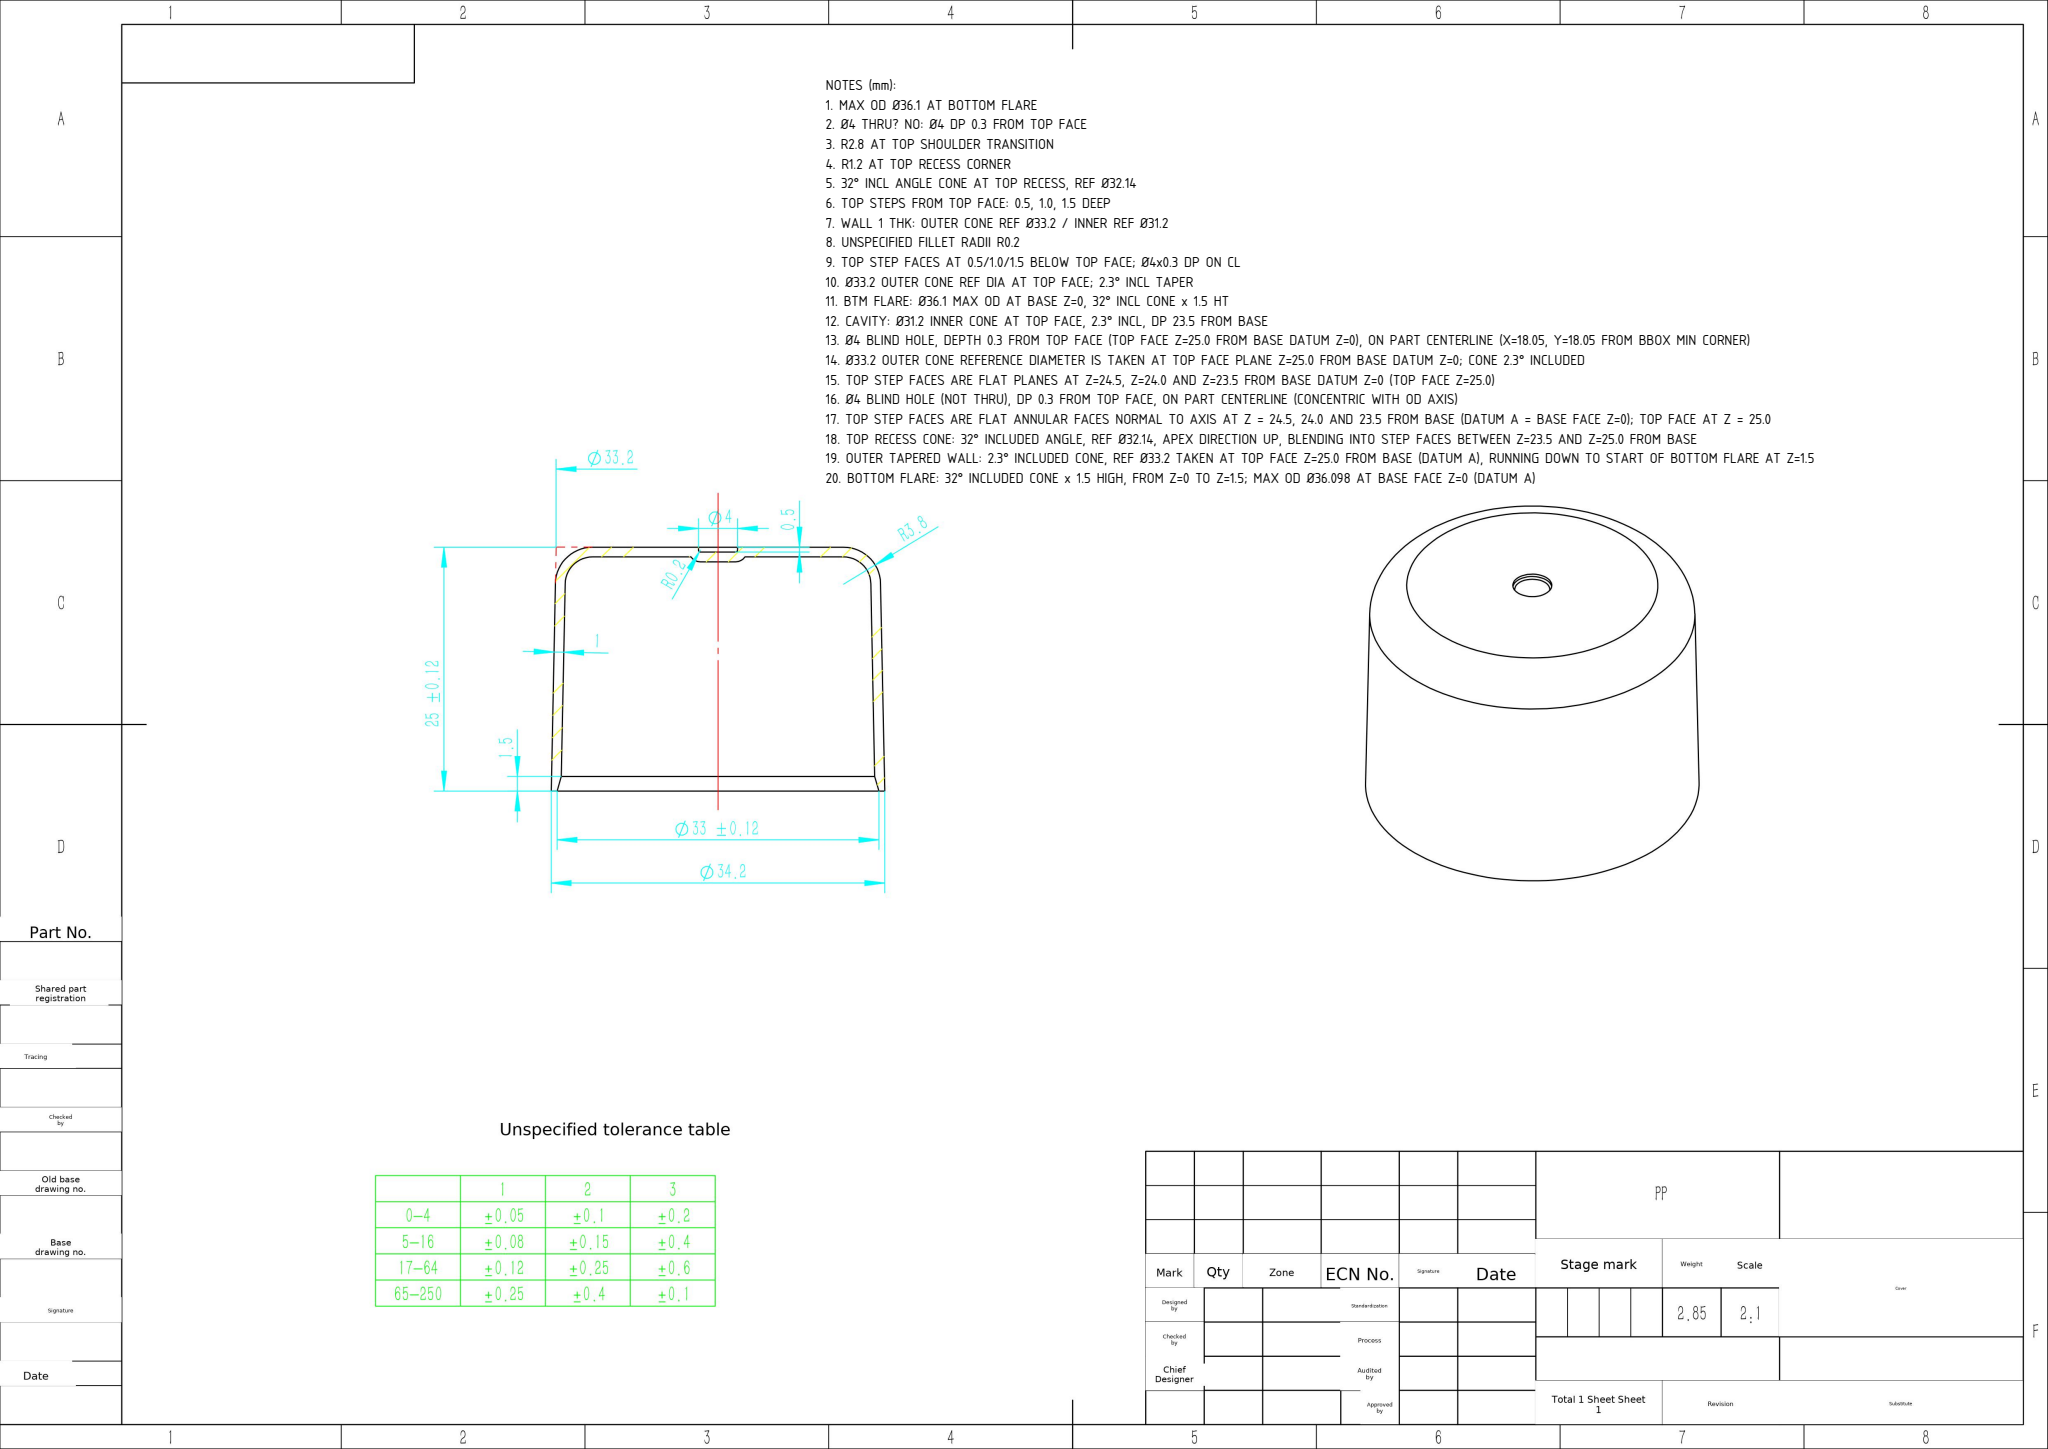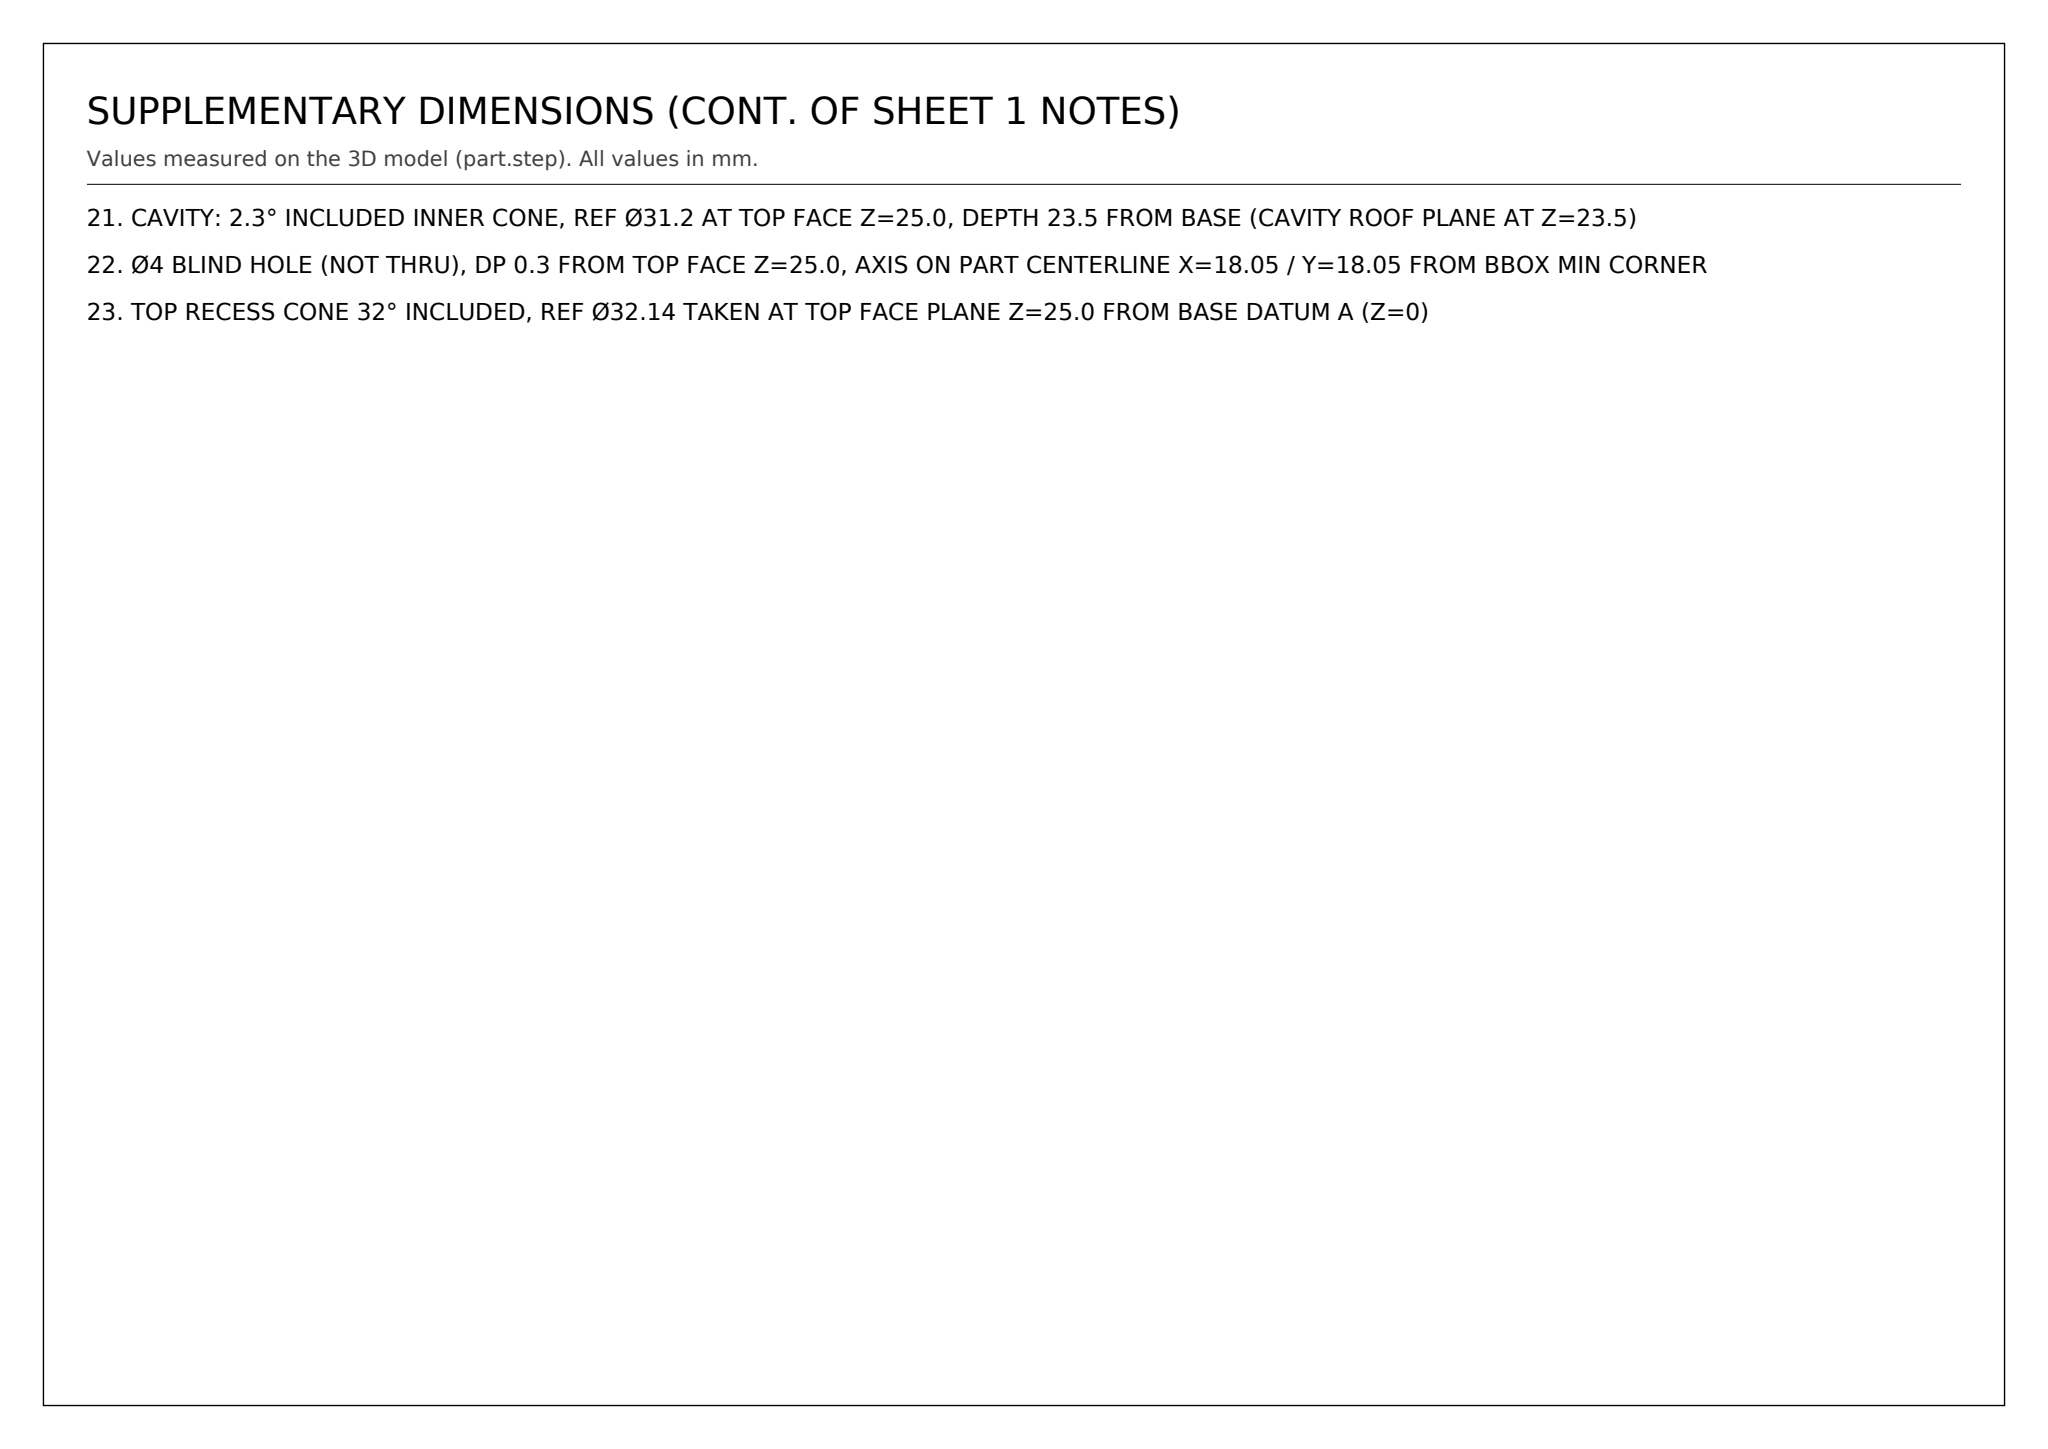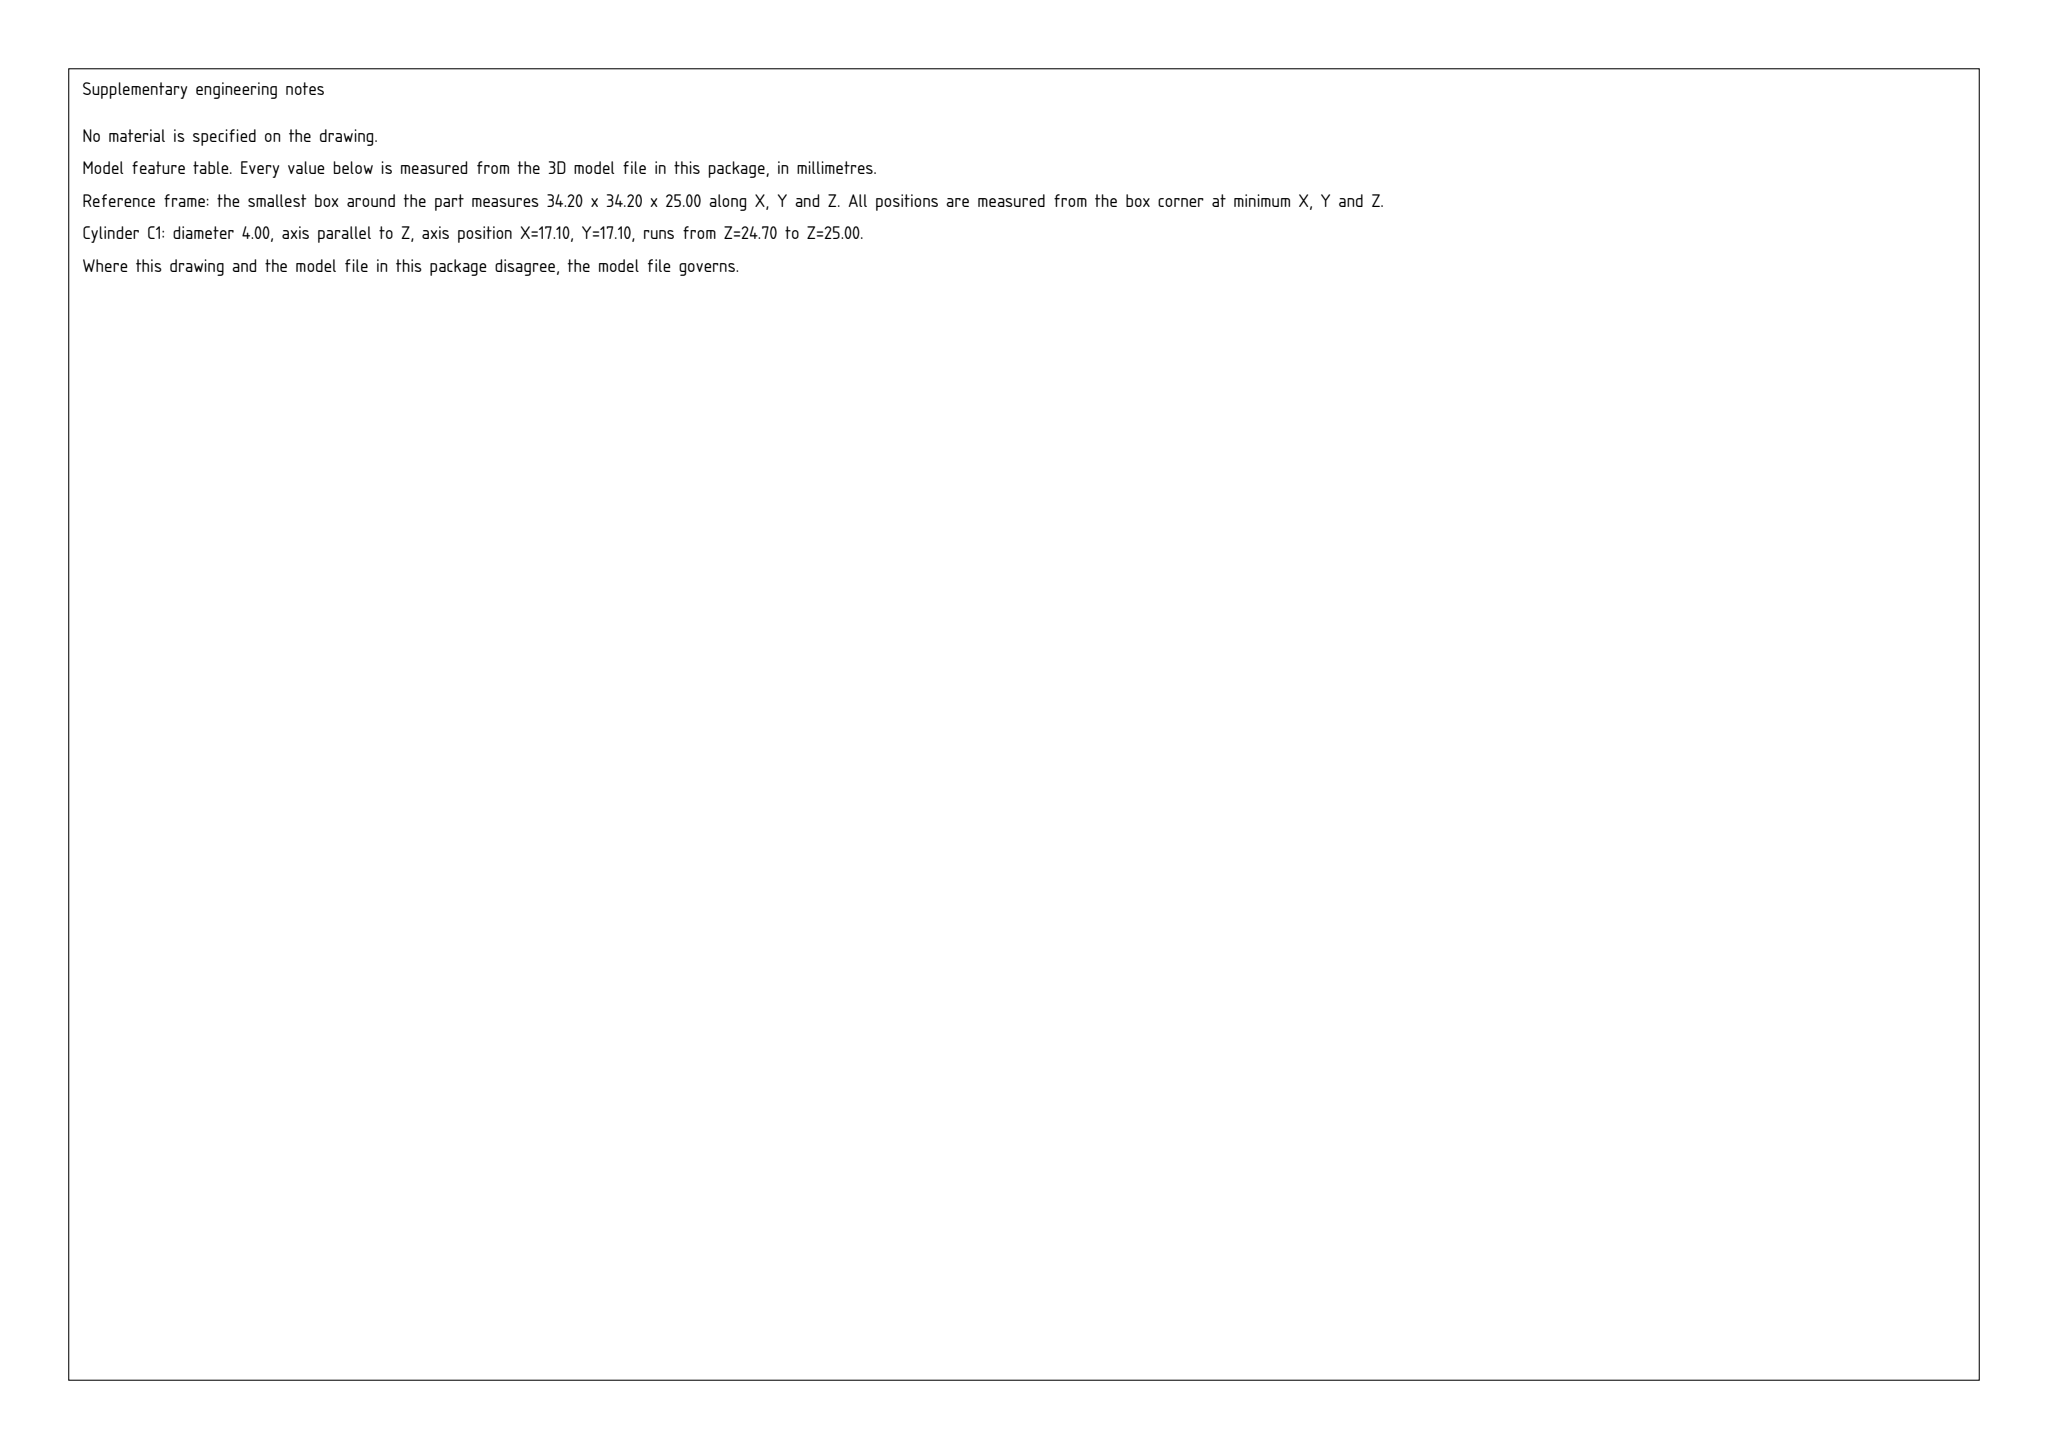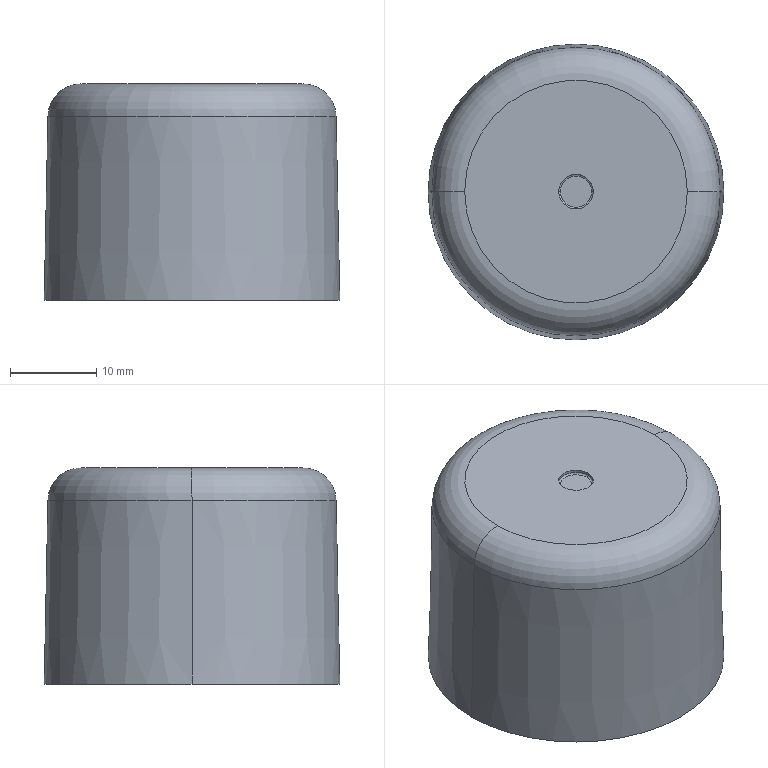Part | SolidWorks | mm | 1 solid | 21 faces | box 34.2 x 34.2 x 25 mm | volume 3165 mm3 | torus 8 | cone 6 | plane 5 | cylinder 2 | commonest cylinder face diameters 4 x2
Drawing notes:
MAX OD Ø36.1 AT BOTTOM FLARE | from the solid: bbox_xyz X/Y = 36.098 at flared bottom
Ø4 THRU? NO: Ø4 DP 0.3 FROM TOP FACE | from the solid: cylinder dia 4.0, axis z, length 0.3 at top (z=25)
R2.8 AT TOP SHOULDER TRANSITION | from the solid: fillet_radii [2.8, 2]
R1.2 AT TOP RECESS CORNER | from the solid: fillet_radii [1.2, 2]
32° INCL ANGLE CONE AT TOP RECESS, REF Ø32.14 | from the solid: cones [32.0, 32.14, 2]
TOP STEPS FROM TOP FACE: 0.5, 1.0, 1.5 DEEP | from the solid: axis_planes z = 24.5, 24.0, 23.5 vs top face z=25.0
WALL 1 THK: OUTER CONE REF Ø33.2 / INNER REF Ø31.2 | from the solid: cones [2.3, 33.2] and [2.3, 31.2]; dia diff 2 = 2 x 1 wall
UNSPECIFIED FILLET RADII R0.2 | from the solid: fillet_radii smallest [0.2, 2]
TOP STEP FACES AT 0.5/1.0/1.5 BELOW TOP FACE; Ø4x0.3 DP ON CL | from the solid: axis_planes z=25.0 (top), 24.5, 24.0, 23.5; cylinder Ø4 on z axis at (18.05,18.05), length 0.3
Ø33.2 OUTER CONE REF DIA AT TOP FACE; 2.3° INCL TAPER | from the solid: cone 2.3° incl, ref_dia 33.2; Ø34.2 at base = 33.2+2*25*tan(1.15°), so Ø33.2 lies at z=25.0 top plane
BTM FLARE: Ø36.1 MAX OD AT BASE Z=0, 32° INCL CONE x 1.5 HT | from the solid: bbox_xyz 36.098 at z=0 plane; cone 32° incl (ref_dia 32.14); step planes give 1.5 flare height
CAVITY: Ø31.2 INNER CONE AT TOP FACE, 2.3° INCL, DP 23.5 FROM BASE | from the solid: cone 2.3° incl ref_dia 31.2 (=33.2-2x1 wall at top); inner top face plane z=23.5, open to z=0
Ø4 BLIND HOLE, DEPTH 0.3 FROM TOP FACE (TOP FACE Z=25.0 FROM BASE DATUM Z=0), ON PART CENTERLINE (X=18.05, Y=18.05 FROM BBOX MIN CORNER) | from the solid: cylinders[dia,axis,pos_other_axes,length]: [4.0, z, [18.05,18.05], 0.3]; axis_planes z=25.0 and z=0.0
Ø33.2 OUTER CONE REFERENCE DIAMETER IS TAKEN AT TOP FACE PLANE Z=25.0 FROM BASE DATUM Z=0; CONE 2.3° INCLUDED | from the solid: cones[included_angle,ref_dia] = [2.3, 33.2]; axis_planes z=25.0, z=0.0
TOP STEP FACES ARE FLAT PLANES AT Z=24.5, Z=24.0 AND Z=23.5 FROM BASE DATUM Z=0 (TOP FACE Z=25.0) | from the solid: axis_planes[normal_axis,offset]: z=24.5, z=24.0, z=23.5, z=25.0, z=0.0
Ø4 BLIND HOLE (NOT THRU), DP 0.3 FROM TOP FACE, ON PART CENTERLINE (CONCENTRIC WITH OD AXIS) | from the solid: cylinders[dia,axis,pos_other_axes,length]: [4.0,'z',[18.05,18.05],0.3] with bbox 36.098 x 36.098 (hole on axis)
TOP STEP FACES ARE FLAT ANNULAR FACES NORMAL TO AXIS AT Z = 24.5, 24.0 AND 23.5 FROM BASE (DATUM A = BASE FACE Z=0); TOP FACE AT Z = 25.0 | from the solid: axis_planes[normal_axis,offset]: z=0.0, z=23.5, z=24.0, z=24.5, z=25.0
TOP RECESS CONE: 32° INCLUDED ANGLE, REF Ø32.14, APEX DIRECTION UP, BLENDING INTO STEP FACES BETWEEN Z=23.5 AND Z=25.0 FROM BASE | from the solid: cones[included_angle,ref_dia]: [32.0, 32.14]
OUTER TAPERED WALL: 2.3° INCLUDED CONE, REF Ø33.2 TAKEN AT TOP FACE Z=25.0 FROM BASE (DATUM A), RUNNING DOWN TO START OF BOTTOM FLARE AT Z=1.5 | from the solid: cones[included_angle,ref_dia]: [2.3, 33.2]; axis_planes z=0.0 and z=25.0; bbox_xyz height 25.0
BOTTOM FLARE: 32° INCLUDED CONE x 1.5 HIGH, FROM Z=0 TO Z=1.5; MAX OD Ø36.098 AT BASE FACE Z=0 (DATUM A) | from the solid: bbox_xyz [36.098, 36.098, 25.0]; cones [32.0]; axis_planes z=0.0
CAVITY: 2.3° INCLUDED INNER CONE, REF Ø31.2 AT TOP FACE Z=25.0, DEPTH 23.5 FROM BASE (CAVITY ROOF PLANE AT Z=23.5) | from the solid: cones[included_angle,ref_dia]: [2.3, 31.2]; axis_planes z=23.5 and z=25.0
Ø4 BLIND HOLE (NOT THRU), DP 0.3 FROM TOP FACE Z=25.0, AXIS ON PART CENTERLINE X=18.05 / Y=18.05 FROM BBOX MIN CORNER | from the solid: cylinders[dia,axis,pos,length]: 4.0, z-axis, (18.05, 18.05), length 0.3; axis_planes z=25.0 (top face)
TOP RECESS CONE 32° INCLUDED, REF Ø32.14 TAKEN AT TOP FACE PLANE Z=25.0 FROM BASE DATUM A (Z=0) | from the solid: cones[included_angle,ref_dia]: 32.0 / 32.14; axis_planes z=25.0 (top face) and z=0.0 (base datum A)
STEP:
#1=CARTESIAN_POINT('',(15.675,0.,21.256));
#2=VERTEX_POINT('',#1);
#3=CARTESIAN_POINT('',(-15.675,0.,21.256));
#4=VERTEX_POINT('',#3);
#5=CARTESIAN_POINT('',(0.,0.,21.256));
#6=DIRECTION('',(0.,0.,-1.));
#7=DIRECTION('',(-1.,0.,0.));
#8=AXIS2_PLACEMENT_3D('',#5,#6,#7);
#9=CIRCLE('',#8,15.675);
#10=EDGE_CURVE('',#2,#4,#9,.T.);
#11=ORIENTED_EDGE('',*,*,#10,.F.);
#12=CARTESIAN_POINT('',(16.07,0.,1.5));
#13=VERTEX_POINT('',#12);
#14=CARTESIAN_POINT('',(15.6,0.,24.98));
#15=DIRECTION('',(0.02,0.,-0.9998));
#16=VECTOR('',#15,1000.);
#17=LINE('',#14,#16);
#18=EDGE_CURVE('',#2,#13,#17,.T.);
#19=ORIENTED_EDGE('',*,*,#18,.T.);
#20=CARTESIAN_POINT('',(-16.07,0.,1.5));
#21=VERTEX_POINT('',#20);
#22=CARTESIAN_POINT('',(0.,0.,1.5));
#23=DIRECTION('',(0.,0.,-1.));
#24=DIRECTION('',(-1.,0.,0.));
#25=AXIS2_PLACEMENT_3D('',#22,#23,#24);
#26=CIRCLE('',#25,16.07);
#27=EDGE_CURVE('',#13,#21,#26,.T.);
#28=ORIENTED_EDGE('',*,*,#27,.T.);
#29=CARTESIAN_POINT('',(-15.6,0.,24.98));
#30=DIRECTION('',(-0.02,0.,-0.9998));
#31=VECTOR('',#30,1000.);
#32=LINE('',#29,#31);
#33=EDGE_CURVE('',#4,#21,#32,.T.);
#34=ORIENTED_EDGE('',*,*,#33,.F.);
#35=EDGE_LOOP('',(#11,#19,#28,#34));
#36=FACE_OUTER_BOUND('',#35,.T.);
#37=CARTESIAN_POINT('',(0.,0.,24.98));
#38=DIRECTION('',(0.,0.,-1.));
#39=DIRECTION('',(-1.,0.,0.));
#40=AXIS2_PLACEMENT_3D('',#37,#38,#39);
#41=CONICAL_SURFACE('',#40,15.6,0.02);
#42=ADVANCED_FACE('',(#36),#41,.F.);
#43=ORIENTED_EDGE('',*,*,#10,.T.);
#44=CARTESIAN_POINT('',(-12.875,0.,24.));
#45=VERTEX_POINT('',#44);
#46=CARTESIAN_POINT('',(-12.875,0.,21.2));
#47=DIRECTION('',(0.,1.,0.));
#48=DIRECTION('',(-1.,0.,0.));
#49=AXIS2_PLACEMENT_3D('',#46,#47,#48);
#50=CIRCLE('',#49,2.8);
#51=EDGE_CURVE('',#4,#45,#50,.T.);
#52=ORIENTED_EDGE('',*,*,#51,.T.);
#53=CARTESIAN_POINT('',(12.875,0.,24.));
#54=VERTEX_POINT('',#53);
#55=CARTESIAN_POINT('',(0.,0.,24.));
#56=DIRECTION('',(0.,0.,1.));
#57=DIRECTION('',(1.,0.,0.));
#58=AXIS2_PLACEMENT_3D('',#55,#56,#57);
#59=CIRCLE('',#58,12.875);
#60=EDGE_CURVE('',#45,#54,#59,.T.);
#61=ORIENTED_EDGE('',*,*,#60,.T.);
#62=CARTESIAN_POINT('',(12.875,0.,21.2));
#63=DIRECTION('',(0.,-1.,0.));
#64=DIRECTION('',(0.,0.,-1.));
#65=AXIS2_PLACEMENT_3D('',#62,#63,#64);
#66=CIRCLE('',#65,2.8);
#67=EDGE_CURVE('',#2,#54,#66,.T.);
#68=ORIENTED_EDGE('',*,*,#67,.F.);
#69=EDGE_LOOP('',(#43,#52,#61,#68));
#70=FACE_OUTER_BOUND('',#69,.T.);
#71=CARTESIAN_POINT('',(0.,0.,21.2));
#72=DIRECTION('',(0.,0.,1.));
#73=DIRECTION('',(1.,0.,0.));
#74=AXIS2_PLACEMENT_3D('',#71,#72,#73);
#75=TOROIDAL_SURFACE('',#74,12.875,2.8);
#76=ADVANCED_FACE('',(#70),#75,.F.);
#77=CARTESIAN_POINT('',(1.8,0.,23.5));
#78=VERTEX_POINT('',#77);
#79=CARTESIAN_POINT('',(-1.8,0.,23.5));
#80=VERTEX_POINT('',#79);
#81=CARTESIAN_POINT('',(0.,0.,23.5));
#82=DIRECTION('',(0.,0.,1.));
#83=DIRECTION('',(1.,0.,0.));
#84=AXIS2_PLACEMENT_3D('',#81,#82,#83);
#85=CIRCLE('',#84,1.8);
#86=EDGE_CURVE('',#78,#80,#85,.T.);
#87=ORIENTED_EDGE('',*,*,#86,.T.);
#88=CARTESIAN_POINT('',(-2.775,0.,24.));
#89=VERTEX_POINT('',#88);
#90=CARTESIAN_POINT('',(-1.8,0.,24.7));
#91=DIRECTION('',(0.,1.,0.));
#92=DIRECTION('',(-1.,0.,0.));
#93=AXIS2_PLACEMENT_3D('',#90,#91,#92);
#94=CIRCLE('',#93,1.2);
#95=EDGE_CURVE('',#80,#89,#94,.T.);
#96=ORIENTED_EDGE('',*,*,#95,.T.);
#97=CARTESIAN_POINT('',(2.775,0.,24.));
#98=VERTEX_POINT('',#97);
#99=CARTESIAN_POINT('',(0.,0.,24.));
#100=DIRECTION('',(0.,0.,-1.));
#101=DIRECTION('',(1.,0.,0.));
#102=AXIS2_PLACEMENT_3D('',#99,#100,#101);
#103=CIRCLE('',#102,2.775);
#104=EDGE_CURVE('',#89,#98,#103,.T.);
#105=ORIENTED_EDGE('',*,*,#104,.T.);
#106=CARTESIAN_POINT('',(1.8,0.,24.7));
#107=DIRECTION('',(0.,-1.,0.));
#108=DIRECTION('',(0.,0.,-1.));
#109=AXIS2_PLACEMENT_3D('',#106,#107,#108);
#110=CIRCLE('',#109,1.2);
#111=EDGE_CURVE('',#78,#98,#110,.T.);
#112=ORIENTED_EDGE('',*,*,#111,.F.);
#113=EDGE_LOOP('',(#87,#96,#105,#112));
#114=FACE_OUTER_BOUND('',#113,.T.);
#115=CARTESIAN_POINT('',(0.,0.,24.7));
#116=DIRECTION('',(0.,0.,1.));
#117=DIRECTION('',(1.,0.,0.));
#118=AXIS2_PLACEMENT_3D('',#115,#116,#117);
#119=TOROIDAL_SURFACE('',#118,1.8,1.2);
#120=ADVANCED_FACE('',(#114),#119,.T.);
#121=ORIENTED_EDGE('',*,*,#27,.F.);
#122=CARTESIAN_POINT('',(16.5,0.,0.));
#123=VERTEX_POINT('',#122);
#124=CARTESIAN_POINT('',(16.07,0.,1.5));
#125=DIRECTION('',(0.2757,0.,-0.9612));
#126=VECTOR('',#125,1000.);
#127=LINE('',#124,#126);
#128=EDGE_CURVE('',#13,#123,#127,.T.);
#129=ORIENTED_EDGE('',*,*,#128,.T.);
#130=CARTESIAN_POINT('',(-16.5,0.,0.));
#131=VERTEX_POINT('',#130);
#132=CARTESIAN_POINT('',(0.,0.,0.));
#133=DIRECTION('',(0.,0.,-1.));
#134=DIRECTION('',(-1.,0.,0.));
#135=AXIS2_PLACEMENT_3D('',#132,#133,#134);
#136=CIRCLE('',#135,16.5);
#137=EDGE_CURVE('',#123,#131,#136,.T.);
#138=ORIENTED_EDGE('',*,*,#137,.T.);
#139=CARTESIAN_POINT('',(-16.07,0.,1.5));
#140=DIRECTION('',(-0.2757,0.,-0.9612));
#141=VECTOR('',#140,1000.);
#142=LINE('',#139,#141);
#143=EDGE_CURVE('',#21,#131,#142,.T.);
#144=ORIENTED_EDGE('',*,*,#143,.F.);
#145=EDGE_LOOP('',(#121,#129,#138,#144));
#146=FACE_OUTER_BOUND('',#145,.T.);
#147=CARTESIAN_POINT('',(0.,0.,1.5));
#148=DIRECTION('',(0.,0.,-1.));
#149=DIRECTION('',(-1.,0.,0.));
#150=AXIS2_PLACEMENT_3D('',#147,#148,#149);
#151=CONICAL_SURFACE('',#150,16.07,0.2793);
#152=ADVANCED_FACE('',(#146),#151,.F.);
#153=CARTESIAN_POINT('',(-1.8,0.,24.5));
#154=VERTEX_POINT('',#153);
#155=CARTESIAN_POINT('',(1.8,0.,24.5));
#156=VERTEX_POINT('',#155);
#157=CARTESIAN_POINT('',(0.,0.,24.5));
#158=DIRECTION('',(0.,0.,1.));
#159=DIRECTION('',(1.,0.,0.));
#160=AXIS2_PLACEMENT_3D('',#157,#158,#159);
#161=CIRCLE('',#160,1.8);
#162=EDGE_CURVE('',#154,#156,#161,.T.);
#163=ORIENTED_EDGE('',*,*,#162,.F.);
#164=CARTESIAN_POINT('',(-2.,0.,24.7));
#165=VERTEX_POINT('',#164);
#166=CARTESIAN_POINT('',(-1.8,0.,24.7));
#167=DIRECTION('',(0.,1.,0.));
#168=DIRECTION('',(-1.,0.,0.));
#169=AXIS2_PLACEMENT_3D('',#166,#167,#168);
#170=CIRCLE('',#169,0.2);
#171=EDGE_CURVE('',#154,#165,#170,.T.);
#172=ORIENTED_EDGE('',*,*,#171,.T.);
#173=CARTESIAN_POINT('',(2.,0.,24.7));
#174=VERTEX_POINT('',#173);
#175=CARTESIAN_POINT('',(0.,0.,24.7));
#176=DIRECTION('',(0.,0.,-1.));
#177=DIRECTION('',(1.,0.,0.));
#178=AXIS2_PLACEMENT_3D('',#175,#176,#177);
#179=CIRCLE('',#178,2.);
#180=EDGE_CURVE('',#174,#165,#179,.T.);
#181=ORIENTED_EDGE('',*,*,#180,.F.);
#182=CARTESIAN_POINT('',(1.8,0.,24.7));
#183=DIRECTION('',(0.,-1.,0.));
#184=DIRECTION('',(0.,0.,-1.));
#185=AXIS2_PLACEMENT_3D('',#182,#183,#184);
#186=CIRCLE('',#185,0.2);
#187=EDGE_CURVE('',#156,#174,#186,.T.);
#188=ORIENTED_EDGE('',*,*,#187,.F.);
#189=EDGE_LOOP('',(#163,#172,#181,#188));
#190=FACE_OUTER_BOUND('',#189,.T.);
#191=CARTESIAN_POINT('',(0.,0.,24.7));
#192=DIRECTION('',(0.,0.,1.));
#193=DIRECTION('',(1.,0.,0.));
#194=AXIS2_PLACEMENT_3D('',#191,#192,#193);
#195=TOROIDAL_SURFACE('',#194,1.8,0.2);
#196=ADVANCED_FACE('',(#190),#195,.F.);
#197=ORIENTED_EDGE('',*,*,#180,.T.);
#198=CARTESIAN_POINT('',(-2.,0.,25.));
#199=VERTEX_POINT('',#198);
#200=CARTESIAN_POINT('',(-2.,0.,24.5));
#201=DIRECTION('',(0.,0.,1.));
#202=VECTOR('',#201,1000.);
#203=LINE('',#200,#202);
#204=EDGE_CURVE('',#165,#199,#203,.T.);
#205=ORIENTED_EDGE('',*,*,#204,.T.);
#206=CARTESIAN_POINT('',(2.,0.,25.));
#207=VERTEX_POINT('',#206);
#208=CARTESIAN_POINT('',(0.,0.,25.));
#209=DIRECTION('',(0.,0.,1.));
#210=DIRECTION('',(1.,0.,0.));
#211=AXIS2_PLACEMENT_3D('',#208,#209,#210);
#212=CIRCLE('',#211,2.);
#213=EDGE_CURVE('',#199,#207,#212,.T.);
#214=ORIENTED_EDGE('',*,*,#213,.T.);
#215=CARTESIAN_POINT('',(2.,0.,24.5));
#216=DIRECTION('',(0.,0.,1.));
#217=VECTOR('',#216,1000.);
#218=LINE('',#215,#217);
#219=EDGE_CURVE('',#174,#207,#218,.T.);
#220=ORIENTED_EDGE('',*,*,#219,.F.);
#221=EDGE_LOOP('',(#197,#205,#214,#220));
#222=FACE_OUTER_BOUND('',#221,.T.);
#223=CARTESIAN_POINT('',(0.,0.,24.5));
#224=DIRECTION('',(0.,0.,1.));
#225=DIRECTION('',(1.,0.,0.));
#226=AXIS2_PLACEMENT_3D('',#223,#224,#225);
#227=CYLINDRICAL_SURFACE('',#226,2.);
#228=ADVANCED_FACE('',(#222),#227,.F.);
#229=CARTESIAN_POINT('',(-16.674,0.,21.276));
#230=VERTEX_POINT('',#229);
#231=CARTESIAN_POINT('',(16.674,0.,21.276));
#232=VERTEX_POINT('',#231);
#233=CARTESIAN_POINT('',(0.,0.,21.276));
#234=DIRECTION('',(0.,0.,-1.));
#235=DIRECTION('',(-1.,0.,0.));
#236=AXIS2_PLACEMENT_3D('',#233,#234,#235);
#237=CIRCLE('',#236,16.674);
#238=EDGE_CURVE('',#230,#232,#237,.T.);
#239=ORIENTED_EDGE('',*,*,#238,.F.);
#240=CARTESIAN_POINT('',(-12.875,0.,25.));
#241=VERTEX_POINT('',#240);
#242=CARTESIAN_POINT('',(-12.875,0.,21.2));
#243=DIRECTION('',(0.,1.,0.));
#244=DIRECTION('',(-1.,0.,0.));
#245=AXIS2_PLACEMENT_3D('',#242,#243,#244);
#246=CIRCLE('',#245,3.8);
#247=EDGE_CURVE('',#230,#241,#246,.T.);
#248=ORIENTED_EDGE('',*,*,#247,.T.);
#249=CARTESIAN_POINT('',(12.875,0.,25.));
#250=VERTEX_POINT('',#249);
#251=CARTESIAN_POINT('',(0.,0.,25.));
#252=DIRECTION('',(0.,0.,1.));
#253=DIRECTION('',(1.,0.,0.));
#254=AXIS2_PLACEMENT_3D('',#251,#252,#253);
#255=CIRCLE('',#254,12.875);
#256=EDGE_CURVE('',#250,#241,#255,.T.);
#257=ORIENTED_EDGE('',*,*,#256,.F.);
#258=CARTESIAN_POINT('',(12.875,0.,21.2));
#259=DIRECTION('',(0.,-1.,0.));
#260=DIRECTION('',(0.,0.,-1.));
#261=AXIS2_PLACEMENT_3D('',#258,#259,#260);
#262=CIRCLE('',#261,3.8);
#263=EDGE_CURVE('',#232,#250,#262,.T.);
#264=ORIENTED_EDGE('',*,*,#263,.F.);
#265=EDGE_LOOP('',(#239,#248,#257,#264));
#266=FACE_OUTER_BOUND('',#265,.T.);
#267=CARTESIAN_POINT('',(0.,0.,21.2));
#268=DIRECTION('',(0.,0.,1.));
#269=DIRECTION('',(1.,0.,0.));
#270=AXIS2_PLACEMENT_3D('',#267,#268,#269);
#271=TOROIDAL_SURFACE('',#270,12.875,3.8);
#272=ADVANCED_FACE('',(#266),#271,.T.);
#273=ORIENTED_EDGE('',*,*,#238,.T.);
#274=CARTESIAN_POINT('',(17.1,0.,0.));
#275=VERTEX_POINT('',#274);
#276=CARTESIAN_POINT('',(16.6,0.,25.));
#277=DIRECTION('',(0.02,0.,-0.9998));
#278=VECTOR('',#277,1000.);
#279=LINE('',#276,#278);
#280=EDGE_CURVE('',#232,#275,#279,.T.);
#281=ORIENTED_EDGE('',*,*,#280,.T.);
#282=CARTESIAN_POINT('',(-17.1,0.,0.));
#283=VERTEX_POINT('',#282);
#284=CARTESIAN_POINT('',(0.,0.,0.));
#285=DIRECTION('',(0.,0.,-1.));
#286=DIRECTION('',(-1.,0.,0.));
#287=AXIS2_PLACEMENT_3D('',#284,#285,#286);
#288=CIRCLE('',#287,17.1);
#289=EDGE_CURVE('',#283,#275,#288,.T.);
#290=ORIENTED_EDGE('',*,*,#289,.F.);
#291=CARTESIAN_POINT('',(-16.6,0.,25.));
#292=DIRECTION('',(-0.02,0.,-0.9998));
#293=VECTOR('',#292,1000.);
#294=LINE('',#291,#293);
#295=EDGE_CURVE('',#230,#283,#294,.T.);
#296=ORIENTED_EDGE('',*,*,#295,.F.);
#297=EDGE_LOOP('',(#273,#281,#290,#296));
#298=FACE_OUTER_BOUND('',#297,.T.);
#299=CARTESIAN_POINT('',(0.,0.,25.));
#300=DIRECTION('',(0.,0.,-1.));
#301=DIRECTION('',(-1.,0.,0.));
#302=AXIS2_PLACEMENT_3D('',#299,#300,#301);
#303=CONICAL_SURFACE('',#302,16.6,0.02);
#304=ADVANCED_FACE('',(#298),#303,.T.);
#305=CARTESIAN_POINT('',(0.,0.,25.));
#306=DIRECTION('',(0.,0.,1.));
#307=DIRECTION('',(1.,0.,0.));
#308=AXIS2_PLACEMENT_3D('',#305,#306,#307);
#309=CIRCLE('',#308,2.);
#310=EDGE_CURVE('',#207,#199,#309,.T.);
#311=ORIENTED_EDGE('',*,*,#310,.F.);
#312=ORIENTED_EDGE('',*,*,#213,.F.);
#313=EDGE_LOOP('',(#311,#312));
#314=FACE_BOUND('',#313,.T.);
#315=ORIENTED_EDGE('',*,*,#256,.T.);
#316=CARTESIAN_POINT('',(0.,0.,25.));
#317=DIRECTION('',(0.,0.,1.));
#318=DIRECTION('',(1.,0.,0.));
#319=AXIS2_PLACEMENT_3D('',#316,#317,#318);
#320=CIRCLE('',#319,12.875);
#321=EDGE_CURVE('',#241,#250,#320,.T.);
#322=ORIENTED_EDGE('',*,*,#321,.T.);
#323=EDGE_LOOP('',(#315,#322));
#324=FACE_OUTER_BOUND('',#323,.T.);
#325=CARTESIAN_POINT('',(0.,0.,25.));
#326=DIRECTION('',(0.,0.,1.));
#327=DIRECTION('',(1.,0.,0.));
#328=AXIS2_PLACEMENT_3D('',#325,#326,#327);
#329=PLANE('',#328);
#330=ADVANCED_FACE('',(#314,#324),#329,.T.);
#331=ORIENTED_EDGE('',*,*,#280,.F.);
#332=CARTESIAN_POINT('',(0.,0.,21.276));
#333=DIRECTION('',(0.,0.,-1.));
#334=DIRECTION('',(-1.,0.,0.));
#335=AXIS2_PLACEMENT_3D('',#332,#333,#334);
#336=CIRCLE('',#335,16.674);
#337=EDGE_CURVE('',#232,#230,#336,.T.);
#338=ORIENTED_EDGE('',*,*,#337,.T.);
#339=ORIENTED_EDGE('',*,*,#295,.T.);
#340=CARTESIAN_POINT('',(0.,0.,0.));
#341=DIRECTION('',(0.,0.,-1.));
#342=DIRECTION('',(-1.,0.,0.));
#343=AXIS2_PLACEMENT_3D('',#340,#341,#342);
#344=CIRCLE('',#343,17.1);
#345=EDGE_CURVE('',#275,#283,#344,.T.);
#346=ORIENTED_EDGE('',*,*,#345,.F.);
#347=EDGE_LOOP('',(#331,#338,#339,#346));
#348=FACE_OUTER_BOUND('',#347,.T.);
#349=CARTESIAN_POINT('',(0.,0.,25.));
#350=DIRECTION('',(0.,0.,-1.));
#351=DIRECTION('',(-1.,0.,0.));
#352=AXIS2_PLACEMENT_3D('',#349,#350,#351);
#353=CONICAL_SURFACE('',#352,16.6,0.02);
#354=ADVANCED_FACE('',(#348),#353,.T.);
#355=CARTESIAN_POINT('',(0.,0.,0.));
#356=DIRECTION('',(0.,0.,-1.));
#357=DIRECTION('',(-1.,0.,0.));
#358=AXIS2_PLACEMENT_3D('',#355,#356,#357);
#359=CIRCLE('',#358,16.5);
#360=EDGE_CURVE('',#131,#123,#359,.T.);
#361=ORIENTED_EDGE('',*,*,#360,.F.);
#362=ORIENTED_EDGE('',*,*,#137,.F.);
#363=EDGE_LOOP('',(#361,#362));
#364=FACE_BOUND('',#363,.T.);
#365=ORIENTED_EDGE('',*,*,#289,.T.);
#366=ORIENTED_EDGE('',*,*,#345,.T.);
#367=EDGE_LOOP('',(#365,#366));
#368=FACE_OUTER_BOUND('',#367,.T.);
#369=CARTESIAN_POINT('',(0.,0.,0.));
#370=DIRECTION('',(0.,0.,1.));
#371=DIRECTION('',(1.,0.,0.));
#372=AXIS2_PLACEMENT_3D('',#369,#370,#371);
#373=PLANE('',#372);
#374=ADVANCED_FACE('',(#364,#368),#373,.F.);
#375=ORIENTED_EDGE('',*,*,#247,.F.);
#376=ORIENTED_EDGE('',*,*,#337,.F.);
#377=ORIENTED_EDGE('',*,*,#263,.T.);
#378=ORIENTED_EDGE('',*,*,#321,.F.);
#379=EDGE_LOOP('',(#375,#376,#377,#378));
#380=FACE_OUTER_BOUND('',#379,.T.);
#381=CARTESIAN_POINT('',(0.,0.,21.2));
#382=DIRECTION('',(0.,0.,1.));
#383=DIRECTION('',(1.,0.,0.));
#384=AXIS2_PLACEMENT_3D('',#381,#382,#383);
#385=TOROIDAL_SURFACE('',#384,12.875,3.8);
#386=ADVANCED_FACE('',(#380),#385,.T.);
#387=ORIENTED_EDGE('',*,*,#204,.F.);
#388=CARTESIAN_POINT('',(0.,0.,24.7));
#389=DIRECTION('',(0.,0.,-1.));
#390=DIRECTION('',(1.,0.,0.));
#391=AXIS2_PLACEMENT_3D('',#388,#389,#390);
#392=CIRCLE('',#391,2.);
#393=EDGE_CURVE('',#165,#174,#392,.T.);
#394=ORIENTED_EDGE('',*,*,#393,.T.);
#395=ORIENTED_EDGE('',*,*,#219,.T.);
#396=ORIENTED_EDGE('',*,*,#310,.T.);
#397=EDGE_LOOP('',(#387,#394,#395,#396));
#398=FACE_OUTER_BOUND('',#397,.T.);
#399=CARTESIAN_POINT('',(0.,0.,24.5));
#400=DIRECTION('',(0.,0.,1.));
#401=DIRECTION('',(1.,0.,0.));
#402=AXIS2_PLACEMENT_3D('',#399,#400,#401);
#403=CYLINDRICAL_SURFACE('',#402,2.);
#404=ADVANCED_FACE('',(#398),#403,.F.);
#405=CARTESIAN_POINT('',(0.,0.,24.5));
#406=DIRECTION('',(0.,0.,1.));
#407=DIRECTION('',(1.,0.,0.));
#408=AXIS2_PLACEMENT_3D('',#405,#406,#407);
#409=CIRCLE('',#408,1.8);
#410=EDGE_CURVE('',#156,#154,#409,.T.);
#411=ORIENTED_EDGE('',*,*,#410,.T.);
#412=ORIENTED_EDGE('',*,*,#162,.T.);
#413=EDGE_LOOP('',(#411,#412));
#414=FACE_OUTER_BOUND('',#413,.T.);
#415=CARTESIAN_POINT('',(0.,0.,24.5));
#416=DIRECTION('',(0.,0.,1.));
#417=DIRECTION('',(1.,0.,0.));
#418=AXIS2_PLACEMENT_3D('',#415,#416,#417);
#419=PLANE('',#418);
#420=ADVANCED_FACE('',(#414),#419,.T.);
#421=ORIENTED_EDGE('',*,*,#171,.F.);
#422=ORIENTED_EDGE('',*,*,#410,.F.);
#423=ORIENTED_EDGE('',*,*,#187,.T.);
#424=ORIENTED_EDGE('',*,*,#393,.F.);
#425=EDGE_LOOP('',(#421,#422,#423,#424));
#426=FACE_OUTER_BOUND('',#425,.T.);
#427=CARTESIAN_POINT('',(0.,0.,24.7));
#428=DIRECTION('',(0.,0.,1.));
#429=DIRECTION('',(1.,0.,0.));
#430=AXIS2_PLACEMENT_3D('',#427,#428,#429);
#431=TOROIDAL_SURFACE('',#430,1.8,0.2);
#432=ADVANCED_FACE('',(#426),#431,.F.);
#433=ORIENTED_EDGE('',*,*,#128,.F.);
#434=CARTESIAN_POINT('',(0.,0.,1.5));
#435=DIRECTION('',(0.,0.,-1.));
#436=DIRECTION('',(-1.,0.,0.));
#437=AXIS2_PLACEMENT_3D('',#434,#435,#436);
#438=CIRCLE('',#437,16.07);
#439=EDGE_CURVE('',#21,#13,#438,.T.);
#440=ORIENTED_EDGE('',*,*,#439,.F.);
#441=ORIENTED_EDGE('',*,*,#143,.T.);
#442=ORIENTED_EDGE('',*,*,#360,.T.);
#443=EDGE_LOOP('',(#433,#440,#441,#442));
#444=FACE_OUTER_BOUND('',#443,.T.);
#445=CARTESIAN_POINT('',(0.,0.,1.5));
#446=DIRECTION('',(0.,0.,-1.));
#447=DIRECTION('',(-1.,0.,0.));
#448=AXIS2_PLACEMENT_3D('',#445,#446,#447);
#449=CONICAL_SURFACE('',#448,16.07,0.2793);
#450=ADVANCED_FACE('',(#444),#449,.F.);
#451=ORIENTED_EDGE('',*,*,#86,.F.);
#452=CARTESIAN_POINT('',(0.,0.,23.5));
#453=DIRECTION('',(0.,0.,1.));
#454=DIRECTION('',(1.,0.,0.));
#455=AXIS2_PLACEMENT_3D('',#452,#453,#454);
#456=CIRCLE('',#455,1.8);
#457=EDGE_CURVE('',#80,#78,#456,.T.);
#458=ORIENTED_EDGE('',*,*,#457,.F.);
#459=EDGE_LOOP('',(#451,#458));
#460=FACE_OUTER_BOUND('',#459,.T.);
#461=CARTESIAN_POINT('',(0.,0.,23.5));
#462=DIRECTION('',(0.,0.,1.));
#463=DIRECTION('',(1.,0.,0.));
#464=AXIS2_PLACEMENT_3D('',#461,#462,#463);
#465=PLANE('',#464);
#466=ADVANCED_FACE('',(#460),#465,.F.);
#467=ORIENTED_EDGE('',*,*,#95,.F.);
#468=ORIENTED_EDGE('',*,*,#457,.T.);
#469=ORIENTED_EDGE('',*,*,#111,.T.);
#470=CARTESIAN_POINT('',(0.,0.,24.));
#471=DIRECTION('',(0.,0.,-1.));
#472=DIRECTION('',(1.,0.,0.));
#473=AXIS2_PLACEMENT_3D('',#470,#471,#472);
#474=CIRCLE('',#473,2.775);
#475=EDGE_CURVE('',#98,#89,#474,.T.);
#476=ORIENTED_EDGE('',*,*,#475,.T.);
#477=EDGE_LOOP('',(#467,#468,#469,#476));
#478=FACE_OUTER_BOUND('',#477,.T.);
#479=CARTESIAN_POINT('',(0.,0.,24.7));
#480=DIRECTION('',(0.,0.,1.));
#481=DIRECTION('',(1.,0.,0.));
#482=AXIS2_PLACEMENT_3D('',#479,#480,#481);
#483=TOROIDAL_SURFACE('',#482,1.8,1.2);
#484=ADVANCED_FACE('',(#478),#483,.T.);
#485=CARTESIAN_POINT('',(0.,0.,24.));
#486=DIRECTION('',(0.,0.,1.));
#487=DIRECTION('',(1.,0.,0.));
#488=AXIS2_PLACEMENT_3D('',#485,#486,#487);
#489=CIRCLE('',#488,12.875);
#490=EDGE_CURVE('',#54,#45,#489,.T.);
#491=ORIENTED_EDGE('',*,*,#490,.F.);
#492=ORIENTED_EDGE('',*,*,#60,.F.);
#493=EDGE_LOOP('',(#491,#492));
#494=FACE_OUTER_BOUND('',#493,.T.);
#495=ORIENTED_EDGE('',*,*,#475,.F.);
#496=ORIENTED_EDGE('',*,*,#104,.F.);
#497=EDGE_LOOP('',(#495,#496));
#498=FACE_BOUND('',#497,.T.);
#499=CARTESIAN_POINT('',(0.,0.,24.));
#500=DIRECTION('',(0.,0.,1.));
#501=DIRECTION('',(1.,0.,0.));
#502=AXIS2_PLACEMENT_3D('',#499,#500,#501);
#503=PLANE('',#502);
#504=ADVANCED_FACE('',(#494,#498),#503,.F.);
#505=ORIENTED_EDGE('',*,*,#51,.F.);
#506=CARTESIAN_POINT('',(0.,0.,21.256));
#507=DIRECTION('',(0.,0.,-1.));
#508=DIRECTION('',(-1.,0.,0.));
#509=AXIS2_PLACEMENT_3D('',#506,#507,#508);
#510=CIRCLE('',#509,15.675);
#511=EDGE_CURVE('',#4,#2,#510,.T.);
#512=ORIENTED_EDGE('',*,*,#511,.T.);
#513=ORIENTED_EDGE('',*,*,#67,.T.);
#514=ORIENTED_EDGE('',*,*,#490,.T.);
#515=EDGE_LOOP('',(#505,#512,#513,#514));
#516=FACE_OUTER_BOUND('',#515,.T.);
#517=CARTESIAN_POINT('',(0.,0.,21.2));
#518=DIRECTION('',(0.,0.,1.));
#519=DIRECTION('',(1.,0.,0.));
#520=AXIS2_PLACEMENT_3D('',#517,#518,#519);
#521=TOROIDAL_SURFACE('',#520,12.875,2.8);
#522=ADVANCED_FACE('',(#516),#521,.F.);
#523=ORIENTED_EDGE('',*,*,#18,.F.);
#524=ORIENTED_EDGE('',*,*,#511,.F.);
#525=ORIENTED_EDGE('',*,*,#33,.T.);
#526=ORIENTED_EDGE('',*,*,#439,.T.);
#527=EDGE_LOOP('',(#523,#524,#525,#526));
#528=FACE_OUTER_BOUND('',#527,.T.);
#529=CARTESIAN_POINT('',(0.,0.,24.98));
#530=DIRECTION('',(0.,0.,-1.));
#531=DIRECTION('',(-1.,0.,0.));
#532=AXIS2_PLACEMENT_3D('',#529,#530,#531);
#533=CONICAL_SURFACE('',#532,15.6,0.02);
#534=ADVANCED_FACE('',(#528),#533,.F.);
#535=CLOSED_SHELL('',(#42,#76,#120,#152,#196,#228,#272,#304,#330,#354,#374,#386,#404,#420,#432,#450,#466,#484,#504,#522,#534));
#536=MANIFOLD_SOLID_BREP('',#535);
#537=CARTESIAN_POINT('',(0.,0.,0.));
#538=DIRECTION('',(0.,0.,1.));
#539=DIRECTION('',(1.,0.,0.));
#540=AXIS2_PLACEMENT_3D('',#537,#538,#539);
#541=(LENGTH_UNIT()NAMED_UNIT(*)SI_UNIT(.MILLI.,.METRE.));
#542=UNCERTAINTY_MEASURE_WITH_UNIT(LENGTH_MEASURE(0.00001),#541,'','');
#543=(NAMED_UNIT(*)PLANE_ANGLE_UNIT()SI_UNIT($,.RADIAN.));
#544=(NAMED_UNIT(*)SI_UNIT($,.STERADIAN.)SOLID_ANGLE_UNIT());
#545=(GEOMETRIC_REPRESENTATION_CONTEXT(3)GLOBAL_UNCERTAINTY_ASSIGNED_CONTEXT((#542))GLOBAL_UNIT_ASSIGNED_CONTEXT((#541,#543,#544))REPRESENTATION_CONTEXT('',''));
#546=ADVANCED_BREP_SHAPE_REPRESENTATION('',(#536,#540),#545);